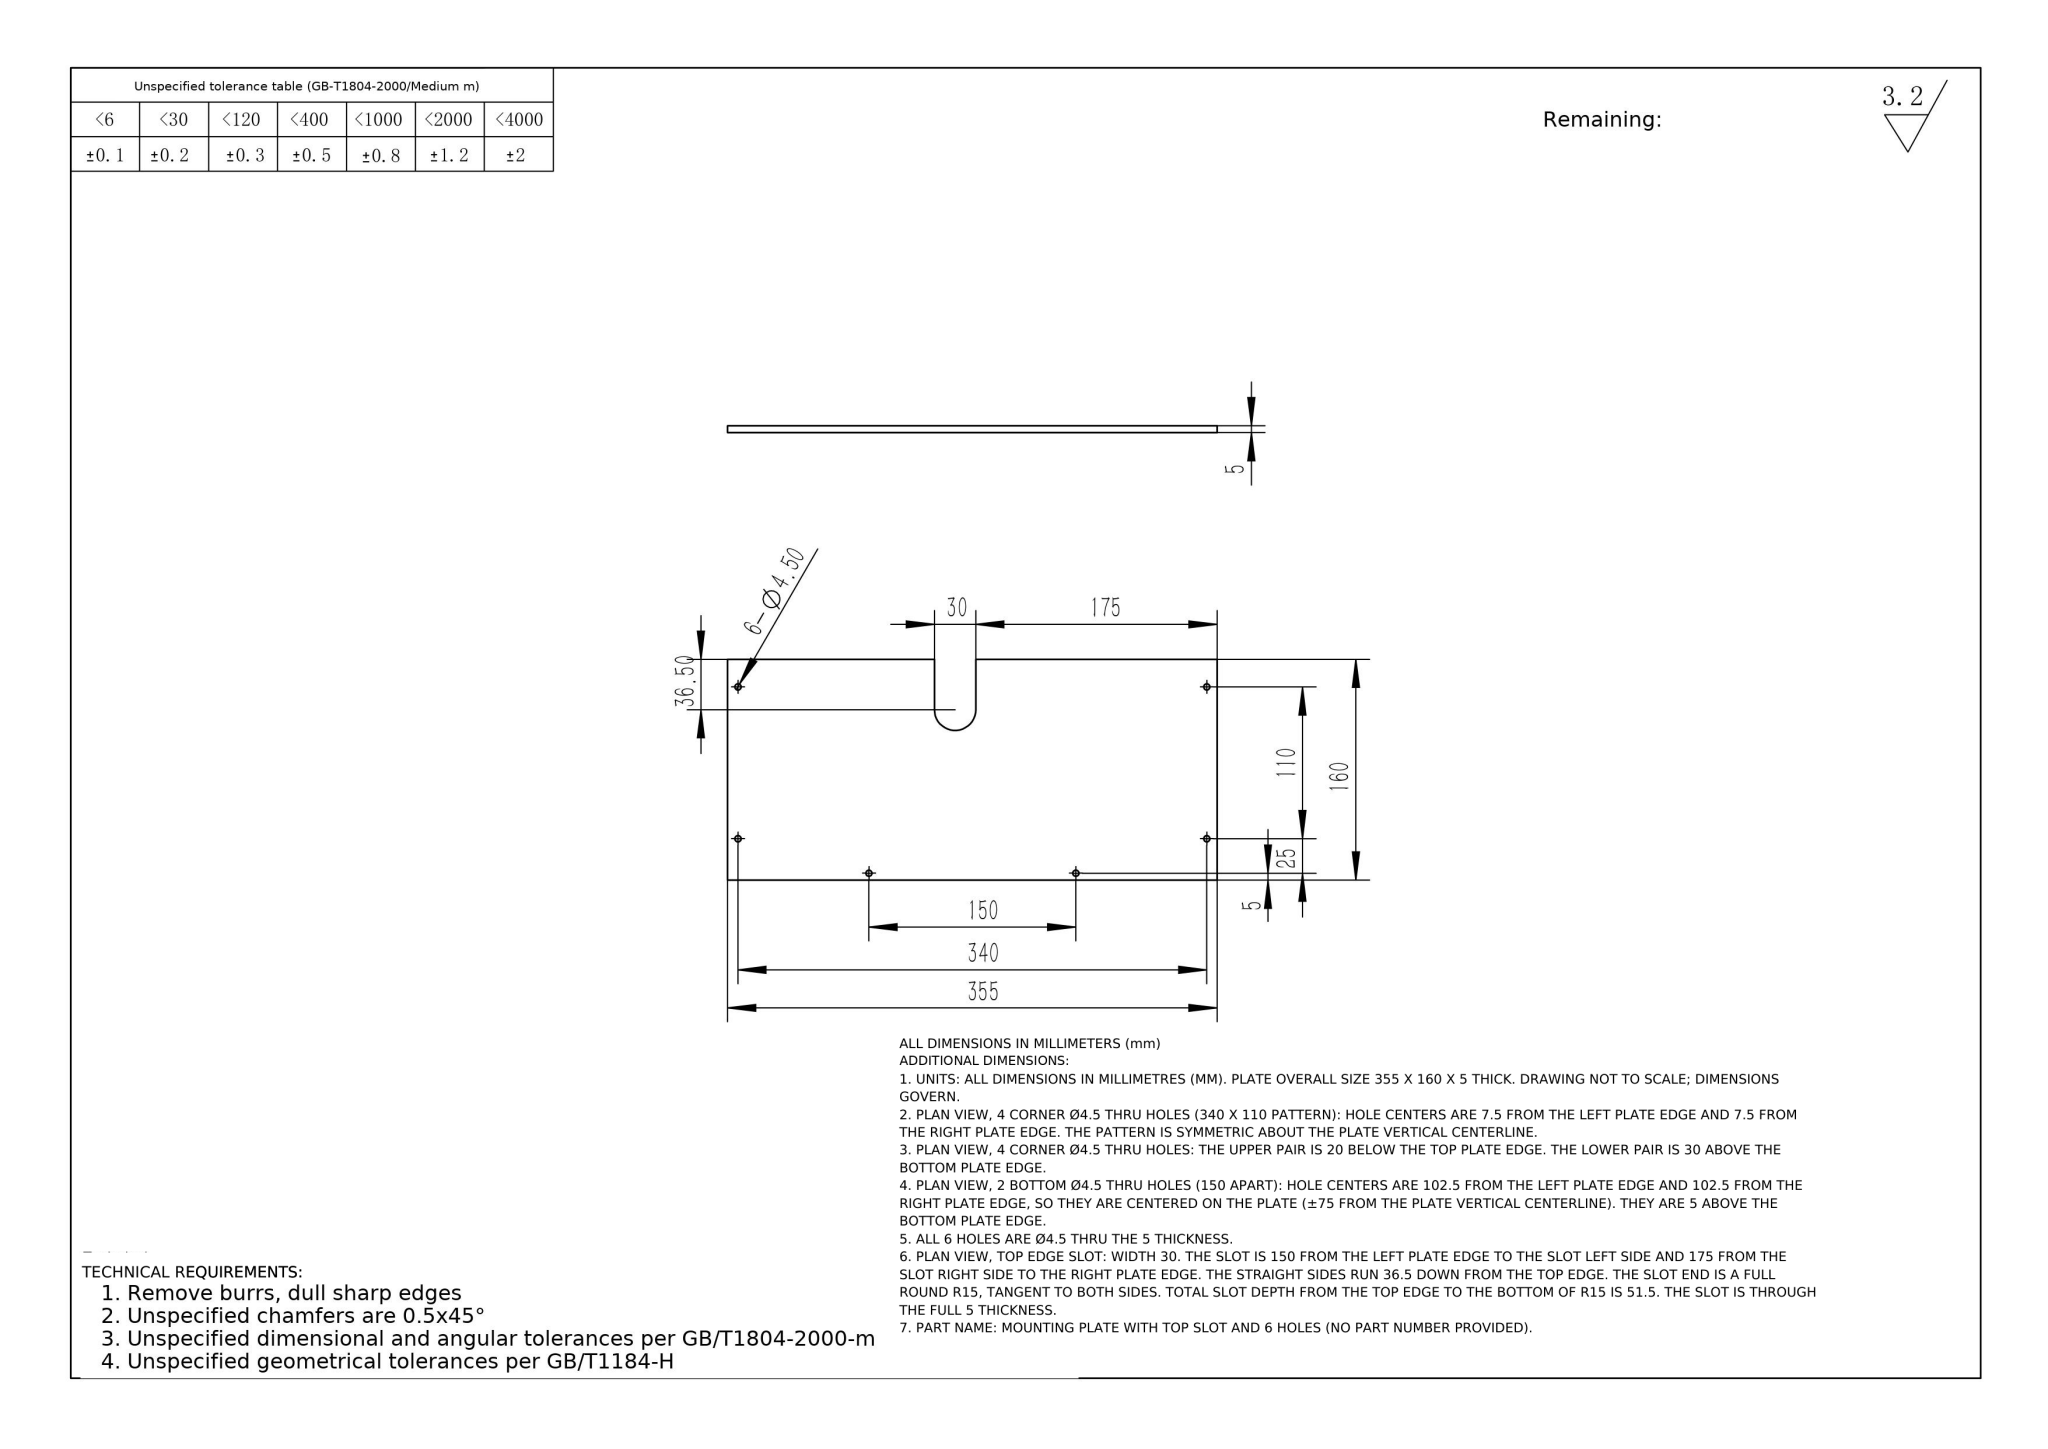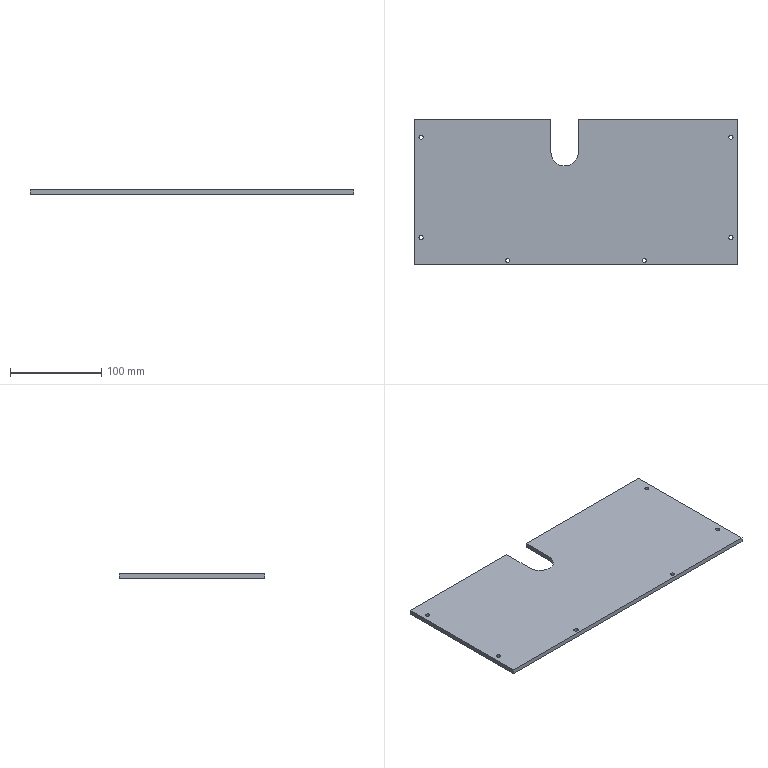Part | NX | mm | 429 | 1 solid | 22 faces | box 355 x 160 x 5 mm | volume 276281 mm3 | cylinder 13 | plane 9 | commonest cylinder face diameters 4.5 x12 30 x1
STEP:
#1=COLOUR_RGB('',1.,1.,1.);
#2=FILL_AREA_STYLE_COLOUR('',#1);
#3=FILL_AREA_STYLE('',(#2));
#4=SURFACE_STYLE_FILL_AREA(#3);
#5=SURFACE_SIDE_STYLE('',(#4));
#6=SURFACE_STYLE_USAGE(.BOTH.,#5);
#7=PRESENTATION_STYLE_ASSIGNMENT((#6));
#8=CARTESIAN_POINT('',(-167.75,-50.,2.5));
#9=VERTEX_POINT('',#8);
#10=CARTESIAN_POINT('',(-172.25,-50.,2.5));
#11=VERTEX_POINT('',#10);
#12=CARTESIAN_POINT('',(-170.,-50.,2.5));
#13=DIRECTION('',(0.,0.,-1.));
#14=DIRECTION('',(-1.,0.,0.));
#15=AXIS2_PLACEMENT_3D('',#12,#13,#14);
#16=CIRCLE('',#15,2.25);
#17=EDGE_CURVE('',#9,#11,#16,.T.);
#18=ORIENTED_EDGE('',*,*,#17,.F.);
#19=CARTESIAN_POINT('',(-167.75,-50.,-2.5));
#20=VERTEX_POINT('',#19);
#21=CARTESIAN_POINT('',(-167.75,-50.,-2.5));
#22=DIRECTION('',(0.,0.,-1.));
#23=VECTOR('',#22,1000.);
#24=LINE('',#21,#23);
#25=EDGE_CURVE('',#9,#20,#24,.T.);
#26=ORIENTED_EDGE('',*,*,#25,.T.);
#27=CARTESIAN_POINT('',(-172.25,-50.,-2.5));
#28=VERTEX_POINT('',#27);
#29=CARTESIAN_POINT('',(-170.,-50.,-2.5));
#30=DIRECTION('',(0.,0.,-1.));
#31=DIRECTION('',(-1.,0.,0.));
#32=AXIS2_PLACEMENT_3D('',#29,#30,#31);
#33=CIRCLE('',#32,2.25);
#34=EDGE_CURVE('',#20,#28,#33,.T.);
#35=ORIENTED_EDGE('',*,*,#34,.T.);
#36=CARTESIAN_POINT('',(-172.25,-50.,-2.5));
#37=DIRECTION('',(0.,0.,-1.));
#38=VECTOR('',#37,1000.);
#39=LINE('',#36,#38);
#40=EDGE_CURVE('',#11,#28,#39,.T.);
#41=ORIENTED_EDGE('',*,*,#40,.F.);
#42=EDGE_LOOP('',(#18,#26,#35,#41));
#43=FACE_OUTER_BOUND('',#42,.T.);
#44=CARTESIAN_POINT('',(-170.,-50.,-2.5));
#45=DIRECTION('',(0.,0.,-1.));
#46=DIRECTION('',(-1.,0.,0.));
#47=AXIS2_PLACEMENT_3D('',#44,#45,#46);
#48=CYLINDRICAL_SURFACE('',#47,2.25);
#49=ADVANCED_FACE('',(#43),#48,.F.);
#50=CARTESIAN_POINT('',(-167.75,60.,2.5));
#51=VERTEX_POINT('',#50);
#52=CARTESIAN_POINT('',(-172.25,60.,2.5));
#53=VERTEX_POINT('',#52);
#54=CARTESIAN_POINT('',(-170.,60.,2.5));
#55=DIRECTION('',(0.,0.,-1.));
#56=DIRECTION('',(-1.,0.,0.));
#57=AXIS2_PLACEMENT_3D('',#54,#55,#56);
#58=CIRCLE('',#57,2.25);
#59=EDGE_CURVE('',#51,#53,#58,.T.);
#60=ORIENTED_EDGE('',*,*,#59,.F.);
#61=CARTESIAN_POINT('',(-167.75,60.,-2.5));
#62=VERTEX_POINT('',#61);
#63=CARTESIAN_POINT('',(-167.75,60.,-2.5));
#64=DIRECTION('',(0.,0.,-1.));
#65=VECTOR('',#64,1000.);
#66=LINE('',#63,#65);
#67=EDGE_CURVE('',#51,#62,#66,.T.);
#68=ORIENTED_EDGE('',*,*,#67,.T.);
#69=CARTESIAN_POINT('',(-172.25,60.,-2.5));
#70=VERTEX_POINT('',#69);
#71=CARTESIAN_POINT('',(-170.,60.,-2.5));
#72=DIRECTION('',(0.,0.,-1.));
#73=DIRECTION('',(-1.,0.,0.));
#74=AXIS2_PLACEMENT_3D('',#71,#72,#73);
#75=CIRCLE('',#74,2.25);
#76=EDGE_CURVE('',#62,#70,#75,.T.);
#77=ORIENTED_EDGE('',*,*,#76,.T.);
#78=CARTESIAN_POINT('',(-172.25,60.,-2.5));
#79=DIRECTION('',(0.,0.,-1.));
#80=VECTOR('',#79,1000.);
#81=LINE('',#78,#80);
#82=EDGE_CURVE('',#53,#70,#81,.T.);
#83=ORIENTED_EDGE('',*,*,#82,.F.);
#84=EDGE_LOOP('',(#60,#68,#77,#83));
#85=FACE_OUTER_BOUND('',#84,.T.);
#86=CARTESIAN_POINT('',(-170.,60.,-2.5));
#87=DIRECTION('',(0.,0.,-1.));
#88=DIRECTION('',(-1.,0.,0.));
#89=AXIS2_PLACEMENT_3D('',#86,#87,#88);
#90=CYLINDRICAL_SURFACE('',#89,2.25);
#91=ADVANCED_FACE('',(#85),#90,.F.);
#92=CARTESIAN_POINT('',(172.25,60.,2.5));
#93=VERTEX_POINT('',#92);
#94=CARTESIAN_POINT('',(167.75,60.,2.5));
#95=VERTEX_POINT('',#94);
#96=CARTESIAN_POINT('',(170.,60.,2.5));
#97=DIRECTION('',(0.,0.,-1.));
#98=DIRECTION('',(-1.,0.,0.));
#99=AXIS2_PLACEMENT_3D('',#96,#97,#98);
#100=CIRCLE('',#99,2.25);
#101=EDGE_CURVE('',#93,#95,#100,.T.);
#102=ORIENTED_EDGE('',*,*,#101,.F.);
#103=CARTESIAN_POINT('',(172.25,60.,-2.5));
#104=VERTEX_POINT('',#103);
#105=CARTESIAN_POINT('',(172.25,60.,-2.5));
#106=DIRECTION('',(0.,0.,-1.));
#107=VECTOR('',#106,1000.);
#108=LINE('',#105,#107);
#109=EDGE_CURVE('',#93,#104,#108,.T.);
#110=ORIENTED_EDGE('',*,*,#109,.T.);
#111=CARTESIAN_POINT('',(167.75,60.,-2.5));
#112=VERTEX_POINT('',#111);
#113=CARTESIAN_POINT('',(170.,60.,-2.5));
#114=DIRECTION('',(0.,0.,-1.));
#115=DIRECTION('',(-1.,0.,0.));
#116=AXIS2_PLACEMENT_3D('',#113,#114,#115);
#117=CIRCLE('',#116,2.25);
#118=EDGE_CURVE('',#104,#112,#117,.T.);
#119=ORIENTED_EDGE('',*,*,#118,.T.);
#120=CARTESIAN_POINT('',(167.75,60.,-2.5));
#121=DIRECTION('',(0.,0.,-1.));
#122=VECTOR('',#121,1000.);
#123=LINE('',#120,#122);
#124=EDGE_CURVE('',#95,#112,#123,.T.);
#125=ORIENTED_EDGE('',*,*,#124,.F.);
#126=EDGE_LOOP('',(#102,#110,#119,#125));
#127=FACE_OUTER_BOUND('',#126,.T.);
#128=CARTESIAN_POINT('',(170.,60.,-2.5));
#129=DIRECTION('',(0.,0.,-1.));
#130=DIRECTION('',(-1.,0.,0.));
#131=AXIS2_PLACEMENT_3D('',#128,#129,#130);
#132=CYLINDRICAL_SURFACE('',#131,2.25);
#133=ADVANCED_FACE('',(#127),#132,.F.);
#134=CARTESIAN_POINT('',(172.25,-50.,2.5));
#135=VERTEX_POINT('',#134);
#136=CARTESIAN_POINT('',(167.75,-50.,2.5));
#137=VERTEX_POINT('',#136);
#138=CARTESIAN_POINT('',(170.,-50.,2.5));
#139=DIRECTION('',(0.,0.,-1.));
#140=DIRECTION('',(-1.,0.,0.));
#141=AXIS2_PLACEMENT_3D('',#138,#139,#140);
#142=CIRCLE('',#141,2.25);
#143=EDGE_CURVE('',#135,#137,#142,.T.);
#144=ORIENTED_EDGE('',*,*,#143,.F.);
#145=CARTESIAN_POINT('',(172.25,-50.,-2.5));
#146=VERTEX_POINT('',#145);
#147=CARTESIAN_POINT('',(172.25,-50.,-2.5));
#148=DIRECTION('',(0.,0.,-1.));
#149=VECTOR('',#148,1000.);
#150=LINE('',#147,#149);
#151=EDGE_CURVE('',#135,#146,#150,.T.);
#152=ORIENTED_EDGE('',*,*,#151,.T.);
#153=CARTESIAN_POINT('',(167.75,-50.,-2.5));
#154=VERTEX_POINT('',#153);
#155=CARTESIAN_POINT('',(170.,-50.,-2.5));
#156=DIRECTION('',(0.,0.,-1.));
#157=DIRECTION('',(-1.,0.,0.));
#158=AXIS2_PLACEMENT_3D('',#155,#156,#157);
#159=CIRCLE('',#158,2.25);
#160=EDGE_CURVE('',#146,#154,#159,.T.);
#161=ORIENTED_EDGE('',*,*,#160,.T.);
#162=CARTESIAN_POINT('',(167.75,-50.,-2.5));
#163=DIRECTION('',(0.,0.,-1.));
#164=VECTOR('',#163,1000.);
#165=LINE('',#162,#164);
#166=EDGE_CURVE('',#137,#154,#165,.T.);
#167=ORIENTED_EDGE('',*,*,#166,.F.);
#168=EDGE_LOOP('',(#144,#152,#161,#167));
#169=FACE_OUTER_BOUND('',#168,.T.);
#170=CARTESIAN_POINT('',(170.,-50.,-2.5));
#171=DIRECTION('',(0.,0.,-1.));
#172=DIRECTION('',(-1.,0.,0.));
#173=AXIS2_PLACEMENT_3D('',#170,#171,#172);
#174=CYLINDRICAL_SURFACE('',#173,2.25);
#175=ADVANCED_FACE('',(#169),#174,.F.);
#176=CARTESIAN_POINT('',(77.25,-75.,2.5));
#177=VERTEX_POINT('',#176);
#178=CARTESIAN_POINT('',(72.75,-75.,2.5));
#179=VERTEX_POINT('',#178);
#180=CARTESIAN_POINT('',(75.,-75.,2.5));
#181=DIRECTION('',(0.,0.,-1.));
#182=DIRECTION('',(-1.,0.,0.));
#183=AXIS2_PLACEMENT_3D('',#180,#181,#182);
#184=CIRCLE('',#183,2.25);
#185=EDGE_CURVE('',#177,#179,#184,.T.);
#186=ORIENTED_EDGE('',*,*,#185,.F.);
#187=CARTESIAN_POINT('',(77.25,-75.,-2.5));
#188=VERTEX_POINT('',#187);
#189=CARTESIAN_POINT('',(77.25,-75.,-2.5));
#190=DIRECTION('',(0.,0.,-1.));
#191=VECTOR('',#190,1000.);
#192=LINE('',#189,#191);
#193=EDGE_CURVE('',#177,#188,#192,.T.);
#194=ORIENTED_EDGE('',*,*,#193,.T.);
#195=CARTESIAN_POINT('',(72.75,-75.,-2.5));
#196=VERTEX_POINT('',#195);
#197=CARTESIAN_POINT('',(75.,-75.,-2.5));
#198=DIRECTION('',(0.,0.,-1.));
#199=DIRECTION('',(-1.,0.,0.));
#200=AXIS2_PLACEMENT_3D('',#197,#198,#199);
#201=CIRCLE('',#200,2.25);
#202=EDGE_CURVE('',#188,#196,#201,.T.);
#203=ORIENTED_EDGE('',*,*,#202,.T.);
#204=CARTESIAN_POINT('',(72.75,-75.,-2.5));
#205=DIRECTION('',(0.,0.,-1.));
#206=VECTOR('',#205,1000.);
#207=LINE('',#204,#206);
#208=EDGE_CURVE('',#179,#196,#207,.T.);
#209=ORIENTED_EDGE('',*,*,#208,.F.);
#210=EDGE_LOOP('',(#186,#194,#203,#209));
#211=FACE_OUTER_BOUND('',#210,.T.);
#212=CARTESIAN_POINT('',(75.,-75.,-2.5));
#213=DIRECTION('',(0.,0.,-1.));
#214=DIRECTION('',(-1.,0.,0.));
#215=AXIS2_PLACEMENT_3D('',#212,#213,#214);
#216=CYLINDRICAL_SURFACE('',#215,2.25);
#217=ADVANCED_FACE('',(#211),#216,.F.);
#218=CARTESIAN_POINT('',(-72.75,-75.,2.5));
#219=VERTEX_POINT('',#218);
#220=CARTESIAN_POINT('',(-77.25,-75.,2.5));
#221=VERTEX_POINT('',#220);
#222=CARTESIAN_POINT('',(-75.,-75.,2.5));
#223=DIRECTION('',(0.,0.,-1.));
#224=DIRECTION('',(-1.,0.,0.));
#225=AXIS2_PLACEMENT_3D('',#222,#223,#224);
#226=CIRCLE('',#225,2.25);
#227=EDGE_CURVE('',#219,#221,#226,.T.);
#228=ORIENTED_EDGE('',*,*,#227,.F.);
#229=CARTESIAN_POINT('',(-72.75,-75.,-2.5));
#230=VERTEX_POINT('',#229);
#231=CARTESIAN_POINT('',(-72.75,-75.,-2.5));
#232=DIRECTION('',(0.,0.,-1.));
#233=VECTOR('',#232,1000.);
#234=LINE('',#231,#233);
#235=EDGE_CURVE('',#219,#230,#234,.T.);
#236=ORIENTED_EDGE('',*,*,#235,.T.);
#237=CARTESIAN_POINT('',(-77.25,-75.,-2.5));
#238=VERTEX_POINT('',#237);
#239=CARTESIAN_POINT('',(-75.,-75.,-2.5));
#240=DIRECTION('',(0.,0.,-1.));
#241=DIRECTION('',(-1.,0.,0.));
#242=AXIS2_PLACEMENT_3D('',#239,#240,#241);
#243=CIRCLE('',#242,2.25);
#244=EDGE_CURVE('',#230,#238,#243,.T.);
#245=ORIENTED_EDGE('',*,*,#244,.T.);
#246=CARTESIAN_POINT('',(-77.25,-75.,-2.5));
#247=DIRECTION('',(0.,0.,-1.));
#248=VECTOR('',#247,1000.);
#249=LINE('',#246,#248);
#250=EDGE_CURVE('',#221,#238,#249,.T.);
#251=ORIENTED_EDGE('',*,*,#250,.F.);
#252=EDGE_LOOP('',(#228,#236,#245,#251));
#253=FACE_OUTER_BOUND('',#252,.T.);
#254=CARTESIAN_POINT('',(-75.,-75.,-2.5));
#255=DIRECTION('',(0.,0.,-1.));
#256=DIRECTION('',(-1.,0.,0.));
#257=AXIS2_PLACEMENT_3D('',#254,#255,#256);
#258=CYLINDRICAL_SURFACE('',#257,2.25);
#259=ADVANCED_FACE('',(#253),#258,.F.);
#260=CARTESIAN_POINT('',(-27.5,80.,2.5));
#261=VERTEX_POINT('',#260);
#262=CARTESIAN_POINT('',(-177.5,80.,2.5));
#263=VERTEX_POINT('',#262);
#264=CARTESIAN_POINT('',(-177.5,80.,2.5));
#265=DIRECTION('',(-1.,0.,0.));
#266=VECTOR('',#265,1000.);
#267=LINE('',#264,#266);
#268=EDGE_CURVE('',#261,#263,#267,.T.);
#269=ORIENTED_EDGE('',*,*,#268,.F.);
#270=CARTESIAN_POINT('',(-27.5,80.,-2.5));
#271=VERTEX_POINT('',#270);
#272=CARTESIAN_POINT('',(-27.5,80.,-2.5));
#273=DIRECTION('',(0.,0.,1.));
#274=VECTOR('',#273,1000.);
#275=LINE('',#272,#274);
#276=EDGE_CURVE('',#271,#261,#275,.T.);
#277=ORIENTED_EDGE('',*,*,#276,.F.);
#278=CARTESIAN_POINT('',(-177.5,80.,-2.5));
#279=VERTEX_POINT('',#278);
#280=CARTESIAN_POINT('',(-177.5,80.,-2.5));
#281=DIRECTION('',(-1.,0.,0.));
#282=VECTOR('',#281,1000.);
#283=LINE('',#280,#282);
#284=EDGE_CURVE('',#271,#279,#283,.T.);
#285=ORIENTED_EDGE('',*,*,#284,.T.);
#286=CARTESIAN_POINT('',(-177.5,80.,2.5));
#287=DIRECTION('',(0.,0.,-1.));
#288=VECTOR('',#287,1000.);
#289=LINE('',#286,#288);
#290=EDGE_CURVE('',#263,#279,#289,.T.);
#291=ORIENTED_EDGE('',*,*,#290,.F.);
#292=EDGE_LOOP('',(#269,#277,#285,#291));
#293=FACE_OUTER_BOUND('',#292,.T.);
#294=CARTESIAN_POINT('',(-177.5,80.,2.5));
#295=DIRECTION('',(0.,-1.,0.));
#296=DIRECTION('',(0.,0.,-1.));
#297=AXIS2_PLACEMENT_3D('',#294,#295,#296);
#298=PLANE('',#297);
#299=ADVANCED_FACE('',(#293),#298,.F.);
#300=CARTESIAN_POINT('',(177.5,-80.,-2.5));
#301=VERTEX_POINT('',#300);
#302=CARTESIAN_POINT('',(177.5,80.,-2.5));
#303=VERTEX_POINT('',#302);
#304=CARTESIAN_POINT('',(177.5,-80.,-2.5));
#305=DIRECTION('',(0.,1.,0.));
#306=VECTOR('',#305,1000.);
#307=LINE('',#304,#306);
#308=EDGE_CURVE('',#301,#303,#307,.T.);
#309=ORIENTED_EDGE('',*,*,#308,.T.);
#310=CARTESIAN_POINT('',(177.5,80.,2.5));
#311=VERTEX_POINT('',#310);
#312=CARTESIAN_POINT('',(177.5,80.,2.5));
#313=DIRECTION('',(0.,0.,-1.));
#314=VECTOR('',#313,1000.);
#315=LINE('',#312,#314);
#316=EDGE_CURVE('',#311,#303,#315,.T.);
#317=ORIENTED_EDGE('',*,*,#316,.F.);
#318=CARTESIAN_POINT('',(177.5,-80.,2.5));
#319=VERTEX_POINT('',#318);
#320=CARTESIAN_POINT('',(177.5,-80.,2.5));
#321=DIRECTION('',(0.,1.,0.));
#322=VECTOR('',#321,1000.);
#323=LINE('',#320,#322);
#324=EDGE_CURVE('',#319,#311,#323,.T.);
#325=ORIENTED_EDGE('',*,*,#324,.F.);
#326=CARTESIAN_POINT('',(177.5,-80.,2.5));
#327=DIRECTION('',(0.,0.,-1.));
#328=VECTOR('',#327,1000.);
#329=LINE('',#326,#328);
#330=EDGE_CURVE('',#319,#301,#329,.T.);
#331=ORIENTED_EDGE('',*,*,#330,.T.);
#332=EDGE_LOOP('',(#309,#317,#325,#331));
#333=FACE_OUTER_BOUND('',#332,.T.);
#334=CARTESIAN_POINT('',(177.5,-80.,2.5));
#335=DIRECTION('',(-1.,0.,0.));
#336=DIRECTION('',(0.,0.,1.));
#337=AXIS2_PLACEMENT_3D('',#334,#335,#336);
#338=PLANE('',#337);
#339=ADVANCED_FACE('',(#333),#338,.F.);
#340=CARTESIAN_POINT('',(2.5,80.,-2.5));
#341=VERTEX_POINT('',#340);
#342=CARTESIAN_POINT('',(-177.5,80.,-2.5));
#343=DIRECTION('',(-1.,0.,0.));
#344=VECTOR('',#343,1000.);
#345=LINE('',#342,#344);
#346=EDGE_CURVE('',#303,#341,#345,.T.);
#347=ORIENTED_EDGE('',*,*,#346,.T.);
#348=CARTESIAN_POINT('',(2.5,80.,2.5));
#349=VERTEX_POINT('',#348);
#350=CARTESIAN_POINT('',(2.5,80.,-2.5));
#351=DIRECTION('',(0.,0.,1.));
#352=VECTOR('',#351,1000.);
#353=LINE('',#350,#352);
#354=EDGE_CURVE('',#341,#349,#353,.T.);
#355=ORIENTED_EDGE('',*,*,#354,.T.);
#356=CARTESIAN_POINT('',(-177.5,80.,2.5));
#357=DIRECTION('',(-1.,0.,0.));
#358=VECTOR('',#357,1000.);
#359=LINE('',#356,#358);
#360=EDGE_CURVE('',#311,#349,#359,.T.);
#361=ORIENTED_EDGE('',*,*,#360,.F.);
#362=ORIENTED_EDGE('',*,*,#316,.T.);
#363=EDGE_LOOP('',(#347,#355,#361,#362));
#364=FACE_OUTER_BOUND('',#363,.T.);
#365=CARTESIAN_POINT('',(-177.5,80.,2.5));
#366=DIRECTION('',(0.,-1.,0.));
#367=DIRECTION('',(0.,0.,-1.));
#368=AXIS2_PLACEMENT_3D('',#365,#366,#367);
#369=PLANE('',#368);
#370=ADVANCED_FACE('',(#364),#369,.F.);
#371=CARTESIAN_POINT('',(-177.5,-80.,-2.5));
#372=VERTEX_POINT('',#371);
#373=CARTESIAN_POINT('',(-177.5,-80.,-2.5));
#374=DIRECTION('',(0.,-1.,0.));
#375=VECTOR('',#374,1000.);
#376=LINE('',#373,#375);
#377=EDGE_CURVE('',#279,#372,#376,.T.);
#378=ORIENTED_EDGE('',*,*,#377,.T.);
#379=CARTESIAN_POINT('',(-177.5,-80.,2.5));
#380=VERTEX_POINT('',#379);
#381=CARTESIAN_POINT('',(-177.5,-80.,2.5));
#382=DIRECTION('',(0.,0.,-1.));
#383=VECTOR('',#382,1000.);
#384=LINE('',#381,#383);
#385=EDGE_CURVE('',#380,#372,#384,.T.);
#386=ORIENTED_EDGE('',*,*,#385,.F.);
#387=CARTESIAN_POINT('',(-177.5,-80.,2.5));
#388=DIRECTION('',(0.,-1.,0.));
#389=VECTOR('',#388,1000.);
#390=LINE('',#387,#389);
#391=EDGE_CURVE('',#263,#380,#390,.T.);
#392=ORIENTED_EDGE('',*,*,#391,.F.);
#393=ORIENTED_EDGE('',*,*,#290,.T.);
#394=EDGE_LOOP('',(#378,#386,#392,#393));
#395=FACE_OUTER_BOUND('',#394,.T.);
#396=CARTESIAN_POINT('',(-177.5,-80.,2.5));
#397=DIRECTION('',(1.,0.,0.));
#398=DIRECTION('',(0.,0.,-1.));
#399=AXIS2_PLACEMENT_3D('',#396,#397,#398);
#400=PLANE('',#399);
#401=ADVANCED_FACE('',(#395),#400,.F.);
#402=CARTESIAN_POINT('',(-177.5,-80.,-2.5));
#403=DIRECTION('',(1.,0.,0.));
#404=VECTOR('',#403,1000.);
#405=LINE('',#402,#404);
#406=EDGE_CURVE('',#372,#301,#405,.T.);
#407=ORIENTED_EDGE('',*,*,#406,.T.);
#408=ORIENTED_EDGE('',*,*,#330,.F.);
#409=CARTESIAN_POINT('',(-177.5,-80.,2.5));
#410=DIRECTION('',(1.,0.,0.));
#411=VECTOR('',#410,1000.);
#412=LINE('',#409,#411);
#413=EDGE_CURVE('',#380,#319,#412,.T.);
#414=ORIENTED_EDGE('',*,*,#413,.F.);
#415=ORIENTED_EDGE('',*,*,#385,.T.);
#416=EDGE_LOOP('',(#407,#408,#414,#415));
#417=FACE_OUTER_BOUND('',#416,.T.);
#418=CARTESIAN_POINT('',(-177.5,-80.,2.5));
#419=DIRECTION('',(0.,1.,0.));
#420=DIRECTION('',(0.,0.,1.));
#421=AXIS2_PLACEMENT_3D('',#418,#419,#420);
#422=PLANE('',#421);
#423=ADVANCED_FACE('',(#417),#422,.F.);
#424=CARTESIAN_POINT('',(-170.,-50.,2.5));
#425=DIRECTION('',(0.,0.,-1.));
#426=DIRECTION('',(-1.,0.,0.));
#427=AXIS2_PLACEMENT_3D('',#424,#425,#426);
#428=CIRCLE('',#427,2.25);
#429=EDGE_CURVE('',#11,#9,#428,.T.);
#430=ORIENTED_EDGE('',*,*,#429,.T.);
#431=ORIENTED_EDGE('',*,*,#17,.T.);
#432=EDGE_LOOP('',(#430,#431));
#433=FACE_BOUND('',#432,.T.);
#434=CARTESIAN_POINT('',(-170.,60.,2.5));
#435=DIRECTION('',(0.,0.,-1.));
#436=DIRECTION('',(-1.,0.,0.));
#437=AXIS2_PLACEMENT_3D('',#434,#435,#436);
#438=CIRCLE('',#437,2.25);
#439=EDGE_CURVE('',#53,#51,#438,.T.);
#440=ORIENTED_EDGE('',*,*,#439,.T.);
#441=ORIENTED_EDGE('',*,*,#59,.T.);
#442=EDGE_LOOP('',(#440,#441));
#443=FACE_BOUND('',#442,.T.);
#444=CARTESIAN_POINT('',(170.,60.,2.5));
#445=DIRECTION('',(0.,0.,-1.));
#446=DIRECTION('',(-1.,0.,0.));
#447=AXIS2_PLACEMENT_3D('',#444,#445,#446);
#448=CIRCLE('',#447,2.25);
#449=EDGE_CURVE('',#95,#93,#448,.T.);
#450=ORIENTED_EDGE('',*,*,#449,.T.);
#451=ORIENTED_EDGE('',*,*,#101,.T.);
#452=EDGE_LOOP('',(#450,#451));
#453=FACE_BOUND('',#452,.T.);
#454=CARTESIAN_POINT('',(170.,-50.,2.5));
#455=DIRECTION('',(0.,0.,-1.));
#456=DIRECTION('',(-1.,0.,0.));
#457=AXIS2_PLACEMENT_3D('',#454,#455,#456);
#458=CIRCLE('',#457,2.25);
#459=EDGE_CURVE('',#137,#135,#458,.T.);
#460=ORIENTED_EDGE('',*,*,#459,.T.);
#461=ORIENTED_EDGE('',*,*,#143,.T.);
#462=EDGE_LOOP('',(#460,#461));
#463=FACE_BOUND('',#462,.T.);
#464=CARTESIAN_POINT('',(75.,-75.,2.5));
#465=DIRECTION('',(0.,0.,-1.));
#466=DIRECTION('',(-1.,0.,0.));
#467=AXIS2_PLACEMENT_3D('',#464,#465,#466);
#468=CIRCLE('',#467,2.25);
#469=EDGE_CURVE('',#179,#177,#468,.T.);
#470=ORIENTED_EDGE('',*,*,#469,.T.);
#471=ORIENTED_EDGE('',*,*,#185,.T.);
#472=EDGE_LOOP('',(#470,#471));
#473=FACE_BOUND('',#472,.T.);
#474=CARTESIAN_POINT('',(-75.,-75.,2.5));
#475=DIRECTION('',(0.,0.,-1.));
#476=DIRECTION('',(-1.,0.,0.));
#477=AXIS2_PLACEMENT_3D('',#474,#475,#476);
#478=CIRCLE('',#477,2.25);
#479=EDGE_CURVE('',#221,#219,#478,.T.);
#480=ORIENTED_EDGE('',*,*,#479,.T.);
#481=ORIENTED_EDGE('',*,*,#227,.T.);
#482=EDGE_LOOP('',(#480,#481));
#483=FACE_BOUND('',#482,.T.);
#484=CARTESIAN_POINT('',(-27.5,43.5,2.5));
#485=VERTEX_POINT('',#484);
#486=CARTESIAN_POINT('',(2.5,43.5,2.5));
#487=VERTEX_POINT('',#486);
#488=CARTESIAN_POINT('',(-12.5,43.5,2.5));
#489=DIRECTION('',(0.,0.,1.));
#490=DIRECTION('',(1.,0.,0.));
#491=AXIS2_PLACEMENT_3D('',#488,#489,#490);
#492=CIRCLE('',#491,15.);
#493=EDGE_CURVE('',#485,#487,#492,.T.);
#494=ORIENTED_EDGE('',*,*,#493,.F.);
#495=CARTESIAN_POINT('',(-27.5,43.5,2.5));
#496=DIRECTION('',(0.,-1.,0.));
#497=VECTOR('',#496,1000.);
#498=LINE('',#495,#497);
#499=EDGE_CURVE('',#261,#485,#498,.T.);
#500=ORIENTED_EDGE('',*,*,#499,.F.);
#501=ORIENTED_EDGE('',*,*,#268,.T.);
#502=ORIENTED_EDGE('',*,*,#391,.T.);
#503=ORIENTED_EDGE('',*,*,#413,.T.);
#504=ORIENTED_EDGE('',*,*,#324,.T.);
#505=ORIENTED_EDGE('',*,*,#360,.T.);
#506=CARTESIAN_POINT('',(2.5,43.5,2.5));
#507=DIRECTION('',(0.,1.,0.));
#508=VECTOR('',#507,1000.);
#509=LINE('',#506,#508);
#510=EDGE_CURVE('',#487,#349,#509,.T.);
#511=ORIENTED_EDGE('',*,*,#510,.F.);
#512=EDGE_LOOP('',(#494,#500,#501,#502,#503,#504,#505,#511));
#513=FACE_OUTER_BOUND('',#512,.T.);
#514=CARTESIAN_POINT('',(0.,0.,2.5));
#515=DIRECTION('',(0.,0.,-1.));
#516=DIRECTION('',(-1.,0.,0.));
#517=AXIS2_PLACEMENT_3D('',#514,#515,#516);
#518=PLANE('',#517);
#519=ADVANCED_FACE('',(#433,#443,#453,#463,#473,#483,#513),#518,.F.);
#520=CARTESIAN_POINT('',(-170.,-50.,-2.5));
#521=DIRECTION('',(0.,0.,-1.));
#522=DIRECTION('',(-1.,0.,0.));
#523=AXIS2_PLACEMENT_3D('',#520,#521,#522);
#524=CIRCLE('',#523,2.25);
#525=EDGE_CURVE('',#28,#20,#524,.T.);
#526=ORIENTED_EDGE('',*,*,#525,.F.);
#527=ORIENTED_EDGE('',*,*,#34,.F.);
#528=EDGE_LOOP('',(#526,#527));
#529=FACE_BOUND('',#528,.T.);
#530=CARTESIAN_POINT('',(-170.,60.,-2.5));
#531=DIRECTION('',(0.,0.,-1.));
#532=DIRECTION('',(-1.,0.,0.));
#533=AXIS2_PLACEMENT_3D('',#530,#531,#532);
#534=CIRCLE('',#533,2.25);
#535=EDGE_CURVE('',#70,#62,#534,.T.);
#536=ORIENTED_EDGE('',*,*,#535,.F.);
#537=ORIENTED_EDGE('',*,*,#76,.F.);
#538=EDGE_LOOP('',(#536,#537));
#539=FACE_BOUND('',#538,.T.);
#540=CARTESIAN_POINT('',(170.,60.,-2.5));
#541=DIRECTION('',(0.,0.,-1.));
#542=DIRECTION('',(-1.,0.,0.));
#543=AXIS2_PLACEMENT_3D('',#540,#541,#542);
#544=CIRCLE('',#543,2.25);
#545=EDGE_CURVE('',#112,#104,#544,.T.);
#546=ORIENTED_EDGE('',*,*,#545,.F.);
#547=ORIENTED_EDGE('',*,*,#118,.F.);
#548=EDGE_LOOP('',(#546,#547));
#549=FACE_BOUND('',#548,.T.);
#550=CARTESIAN_POINT('',(170.,-50.,-2.5));
#551=DIRECTION('',(0.,0.,-1.));
#552=DIRECTION('',(-1.,0.,0.));
#553=AXIS2_PLACEMENT_3D('',#550,#551,#552);
#554=CIRCLE('',#553,2.25);
#555=EDGE_CURVE('',#154,#146,#554,.T.);
#556=ORIENTED_EDGE('',*,*,#555,.F.);
#557=ORIENTED_EDGE('',*,*,#160,.F.);
#558=EDGE_LOOP('',(#556,#557));
#559=FACE_BOUND('',#558,.T.);
#560=CARTESIAN_POINT('',(75.,-75.,-2.5));
#561=DIRECTION('',(0.,0.,-1.));
#562=DIRECTION('',(-1.,0.,0.));
#563=AXIS2_PLACEMENT_3D('',#560,#561,#562);
#564=CIRCLE('',#563,2.25);
#565=EDGE_CURVE('',#196,#188,#564,.T.);
#566=ORIENTED_EDGE('',*,*,#565,.F.);
#567=ORIENTED_EDGE('',*,*,#202,.F.);
#568=EDGE_LOOP('',(#566,#567));
#569=FACE_BOUND('',#568,.T.);
#570=CARTESIAN_POINT('',(-75.,-75.,-2.5));
#571=DIRECTION('',(0.,0.,-1.));
#572=DIRECTION('',(-1.,0.,0.));
#573=AXIS2_PLACEMENT_3D('',#570,#571,#572);
#574=CIRCLE('',#573,2.25);
#575=EDGE_CURVE('',#238,#230,#574,.T.);
#576=ORIENTED_EDGE('',*,*,#575,.F.);
#577=ORIENTED_EDGE('',*,*,#244,.F.);
#578=EDGE_LOOP('',(#576,#577));
#579=FACE_BOUND('',#578,.T.);
#580=CARTESIAN_POINT('',(-27.5,43.5,-2.5));
#581=VERTEX_POINT('',#580);
#582=CARTESIAN_POINT('',(-27.5,43.5,-2.5));
#583=DIRECTION('',(0.,-1.,0.));
#584=VECTOR('',#583,1000.);
#585=LINE('',#582,#584);
#586=EDGE_CURVE('',#271,#581,#585,.T.);
#587=ORIENTED_EDGE('',*,*,#586,.T.);
#588=CARTESIAN_POINT('',(2.5,43.5,-2.5));
#589=VERTEX_POINT('',#588);
#590=CARTESIAN_POINT('',(-12.5,43.5,-2.5));
#591=DIRECTION('',(0.,0.,1.));
#592=DIRECTION('',(1.,0.,0.));
#593=AXIS2_PLACEMENT_3D('',#590,#591,#592);
#594=CIRCLE('',#593,15.);
#595=EDGE_CURVE('',#581,#589,#594,.T.);
#596=ORIENTED_EDGE('',*,*,#595,.T.);
#597=CARTESIAN_POINT('',(2.5,43.5,-2.5));
#598=DIRECTION('',(0.,1.,0.));
#599=VECTOR('',#598,1000.);
#600=LINE('',#597,#599);
#601=EDGE_CURVE('',#589,#341,#600,.T.);
#602=ORIENTED_EDGE('',*,*,#601,.T.);
#603=ORIENTED_EDGE('',*,*,#346,.F.);
#604=ORIENTED_EDGE('',*,*,#308,.F.);
#605=ORIENTED_EDGE('',*,*,#406,.F.);
#606=ORIENTED_EDGE('',*,*,#377,.F.);
#607=ORIENTED_EDGE('',*,*,#284,.F.);
#608=EDGE_LOOP('',(#587,#596,#602,#603,#604,#605,#606,#607));
#609=FACE_OUTER_BOUND('',#608,.T.);
#610=CARTESIAN_POINT('',(0.,0.,-2.5));
#611=DIRECTION('',(0.,0.,-1.));
#612=DIRECTION('',(-1.,0.,0.));
#613=AXIS2_PLACEMENT_3D('',#610,#611,#612);
#614=PLANE('',#613);
#615=ADVANCED_FACE('',(#529,#539,#549,#559,#569,#579,#609),#614,.T.);
#616=ORIENTED_EDGE('',*,*,#493,.T.);
#617=CARTESIAN_POINT('',(2.5,43.5,-2.5));
#618=DIRECTION('',(0.,0.,1.));
#619=VECTOR('',#618,1000.);
#620=LINE('',#617,#619);
#621=EDGE_CURVE('',#589,#487,#620,.T.);
#622=ORIENTED_EDGE('',*,*,#621,.F.);
#623=ORIENTED_EDGE('',*,*,#595,.F.);
#624=CARTESIAN_POINT('',(-27.5,43.5,-2.5));
#625=DIRECTION('',(0.,0.,1.));
#626=VECTOR('',#625,1000.);
#627=LINE('',#624,#626);
#628=EDGE_CURVE('',#581,#485,#627,.T.);
#629=ORIENTED_EDGE('',*,*,#628,.T.);
#630=EDGE_LOOP('',(#616,#622,#623,#629));
#631=FACE_OUTER_BOUND('',#630,.T.);
#632=CARTESIAN_POINT('',(-12.5,43.5,-2.5));
#633=DIRECTION('',(0.,0.,1.));
#634=DIRECTION('',(1.,0.,0.));
#635=AXIS2_PLACEMENT_3D('',#632,#633,#634);
#636=CYLINDRICAL_SURFACE('',#635,15.);
#637=ADVANCED_FACE('',(#631),#636,.F.);
#638=ORIENTED_EDGE('',*,*,#499,.T.);
#639=ORIENTED_EDGE('',*,*,#628,.F.);
#640=ORIENTED_EDGE('',*,*,#586,.F.);
#641=ORIENTED_EDGE('',*,*,#276,.T.);
#642=EDGE_LOOP('',(#638,#639,#640,#641));
#643=FACE_OUTER_BOUND('',#642,.T.);
#644=CARTESIAN_POINT('',(-27.5,43.5,-2.5));
#645=DIRECTION('',(-1.,0.,0.));
#646=DIRECTION('',(0.,0.,1.));
#647=AXIS2_PLACEMENT_3D('',#644,#645,#646);
#648=PLANE('',#647);
#649=ADVANCED_FACE('',(#643),#648,.F.);
#650=ORIENTED_EDGE('',*,*,#510,.T.);
#651=ORIENTED_EDGE('',*,*,#354,.F.);
#652=ORIENTED_EDGE('',*,*,#601,.F.);
#653=ORIENTED_EDGE('',*,*,#621,.T.);
#654=EDGE_LOOP('',(#650,#651,#652,#653));
#655=FACE_OUTER_BOUND('',#654,.T.);
#656=CARTESIAN_POINT('',(2.5,43.5,-2.5));
#657=DIRECTION('',(1.,0.,0.));
#658=DIRECTION('',(0.,0.,-1.));
#659=AXIS2_PLACEMENT_3D('',#656,#657,#658);
#660=PLANE('',#659);
#661=ADVANCED_FACE('',(#655),#660,.F.);
#662=ORIENTED_EDGE('',*,*,#235,.F.);
#663=ORIENTED_EDGE('',*,*,#479,.F.);
#664=ORIENTED_EDGE('',*,*,#250,.T.);
#665=ORIENTED_EDGE('',*,*,#575,.T.);
#666=EDGE_LOOP('',(#662,#663,#664,#665));
#667=FACE_OUTER_BOUND('',#666,.T.);
#668=CARTESIAN_POINT('',(-75.,-75.,-2.5));
#669=DIRECTION('',(0.,0.,-1.));
#670=DIRECTION('',(-1.,0.,0.));
#671=AXIS2_PLACEMENT_3D('',#668,#669,#670);
#672=CYLINDRICAL_SURFACE('',#671,2.25);
#673=ADVANCED_FACE('',(#667),#672,.F.);
#674=ORIENTED_EDGE('',*,*,#193,.F.);
#675=ORIENTED_EDGE('',*,*,#469,.F.);
#676=ORIENTED_EDGE('',*,*,#208,.T.);
#677=ORIENTED_EDGE('',*,*,#565,.T.);
#678=EDGE_LOOP('',(#674,#675,#676,#677));
#679=FACE_OUTER_BOUND('',#678,.T.);
#680=CARTESIAN_POINT('',(75.,-75.,-2.5));
#681=DIRECTION('',(0.,0.,-1.));
#682=DIRECTION('',(-1.,0.,0.));
#683=AXIS2_PLACEMENT_3D('',#680,#681,#682);
#684=CYLINDRICAL_SURFACE('',#683,2.25);
#685=ADVANCED_FACE('',(#679),#684,.F.);
#686=ORIENTED_EDGE('',*,*,#151,.F.);
#687=ORIENTED_EDGE('',*,*,#459,.F.);
#688=ORIENTED_EDGE('',*,*,#166,.T.);
#689=ORIENTED_EDGE('',*,*,#555,.T.);
#690=EDGE_LOOP('',(#686,#687,#688,#689));
#691=FACE_OUTER_BOUND('',#690,.T.);
#692=CARTESIAN_POINT('',(170.,-50.,-2.5));
#693=DIRECTION('',(0.,0.,-1.));
#694=DIRECTION('',(-1.,0.,0.));
#695=AXIS2_PLACEMENT_3D('',#692,#693,#694);
#696=CYLINDRICAL_SURFACE('',#695,2.25);
#697=ADVANCED_FACE('',(#691),#696,.F.);
#698=ORIENTED_EDGE('',*,*,#109,.F.);
#699=ORIENTED_EDGE('',*,*,#449,.F.);
#700=ORIENTED_EDGE('',*,*,#124,.T.);
#701=ORIENTED_EDGE('',*,*,#545,.T.);
#702=EDGE_LOOP('',(#698,#699,#700,#701));
#703=FACE_OUTER_BOUND('',#702,.T.);
#704=CARTESIAN_POINT('',(170.,60.,-2.5));
#705=DIRECTION('',(0.,0.,-1.));
#706=DIRECTION('',(-1.,0.,0.));
#707=AXIS2_PLACEMENT_3D('',#704,#705,#706);
#708=CYLINDRICAL_SURFACE('',#707,2.25);
#709=ADVANCED_FACE('',(#703),#708,.F.);
#710=ORIENTED_EDGE('',*,*,#67,.F.);
#711=ORIENTED_EDGE('',*,*,#439,.F.);
#712=ORIENTED_EDGE('',*,*,#82,.T.);
#713=ORIENTED_EDGE('',*,*,#535,.T.);
#714=EDGE_LOOP('',(#710,#711,#712,#713));
#715=FACE_OUTER_BOUND('',#714,.T.);
#716=CARTESIAN_POINT('',(-170.,60.,-2.5));
#717=DIRECTION('',(0.,0.,-1.));
#718=DIRECTION('',(-1.,0.,0.));
#719=AXIS2_PLACEMENT_3D('',#716,#717,#718);
#720=CYLINDRICAL_SURFACE('',#719,2.25);
#721=ADVANCED_FACE('',(#715),#720,.F.);
#722=ORIENTED_EDGE('',*,*,#25,.F.);
#723=ORIENTED_EDGE('',*,*,#429,.F.);
#724=ORIENTED_EDGE('',*,*,#40,.T.);
#725=ORIENTED_EDGE('',*,*,#525,.T.);
#726=EDGE_LOOP('',(#722,#723,#724,#725));
#727=FACE_OUTER_BOUND('',#726,.T.);
#728=CARTESIAN_POINT('',(-170.,-50.,-2.5));
#729=DIRECTION('',(0.,0.,-1.));
#730=DIRECTION('',(-1.,0.,0.));
#731=AXIS2_PLACEMENT_3D('',#728,#729,#730);
#732=CYLINDRICAL_SURFACE('',#731,2.25);
#733=ADVANCED_FACE('',(#727),#732,.F.);
#734=CLOSED_SHELL('',(#49,#91,#133,#175,#217,#259,#299,#339,#370,#401,#423,#519,#615,#637,#649,#661,#673,#685,#697,#709,#721,#733));
#735=MANIFOLD_SOLID_BREP('',#734);
#736=STYLED_ITEM('',(#7),#735);
#737=PRESENTATION_LAYER_ASSIGNMENT('','',(#736));
#738=(LENGTH_UNIT()NAMED_UNIT(*)SI_UNIT(.MILLI.,.METRE.));
#739=UNCERTAINTY_MEASURE_WITH_UNIT(LENGTH_MEASURE(0.00001),#738,'','');
#740=(NAMED_UNIT(*)PLANE_ANGLE_UNIT()SI_UNIT($,.RADIAN.));
#741=(NAMED_UNIT(*)SI_UNIT($,.STERADIAN.)SOLID_ANGLE_UNIT());
#742=(GEOMETRIC_REPRESENTATION_CONTEXT(3)GLOBAL_UNCERTAINTY_ASSIGNED_CONTEXT((#739))GLOBAL_UNIT_ASSIGNED_CONTEXT((#738,#740,#741))REPRESENTATION_CONTEXT('',''));
#743=MECHANICAL_DESIGN_GEOMETRIC_PRESENTATION_REPRESENTATION('',(#736),#742);
#744=COLOUR_RGB('',1.,1.,1.);
#745=FILL_AREA_STYLE_COLOUR('',#744);
#746=FILL_AREA_STYLE('',(#745));
#747=SURFACE_STYLE_FILL_AREA(#746);
#748=SURFACE_SIDE_STYLE('',(#747));
#749=SURFACE_STYLE_USAGE(.BOTH.,#748);
#750=PRESENTATION_STYLE_ASSIGNMENT((#749));
#751=CARTESIAN_POINT('',(0.,0.,0.));
#752=DIRECTION('',(0.,0.,1.));
#753=DIRECTION('',(1.,0.,0.));
#754=AXIS2_PLACEMENT_3D('',#751,#752,#753);
#755=(LENGTH_UNIT()NAMED_UNIT(*)SI_UNIT(.MILLI.,.METRE.));
#756=UNCERTAINTY_MEASURE_WITH_UNIT(LENGTH_MEASURE(0.00001),#755,'','');
#757=(NAMED_UNIT(*)PLANE_ANGLE_UNIT()SI_UNIT($,.RADIAN.));
#758=(NAMED_UNIT(*)SI_UNIT($,.STERADIAN.)SOLID_ANGLE_UNIT());
#759=(GEOMETRIC_REPRESENTATION_CONTEXT(3)GLOBAL_UNCERTAINTY_ASSIGNED_CONTEXT((#756))GLOBAL_UNIT_ASSIGNED_CONTEXT((#755,#757,#758))REPRESENTATION_CONTEXT('',''));
#760=ADVANCED_BREP_SHAPE_REPRESENTATION('',(#735,#754),#759);
#761=STYLED_ITEM('',(#750),#760);
#762=(LENGTH_UNIT()NAMED_UNIT(*)SI_UNIT(.MILLI.,.METRE.));
#763=UNCERTAINTY_MEASURE_WITH_UNIT(LENGTH_MEASURE(0.00001),#762,'','');
#764=(NAMED_UNIT(*)PLANE_ANGLE_UNIT()SI_UNIT($,.RADIAN.));
#765=(NAMED_UNIT(*)SI_UNIT($,.STERADIAN.)SOLID_ANGLE_UNIT());
#766=(GEOMETRIC_REPRESENTATION_CONTEXT(3)GLOBAL_UNCERTAINTY_ASSIGNED_CONTEXT((#763))GLOBAL_UNIT_ASSIGNED_CONTEXT((#762,#764,#765))REPRESENTATION_CONTEXT('',''));
#767=MECHANICAL_DESIGN_GEOMETRIC_PRESENTATION_REPRESENTATION('',(#761),#766);
#768=PRESENTATION_LAYER_ASSIGNMENT('','',(#761));